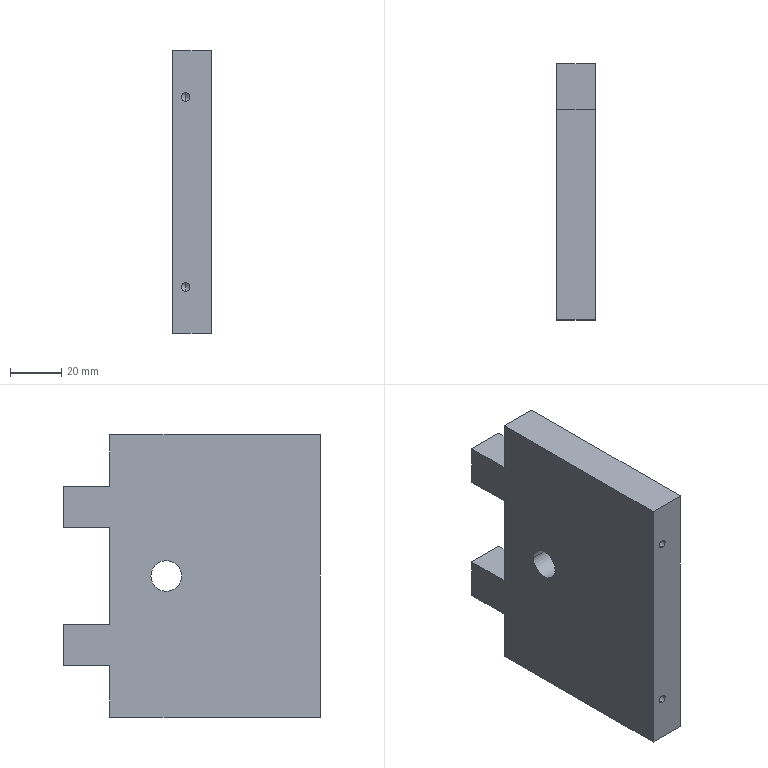Component | SolidWorks | CS021-A10-A002-1 | 1 solid | 32 faces | box 15 x 100 x 110 mm | volume 141686 mm3 | plane 14 | cylinder 10 | cone 8 | commonest cylinder face diameters 4.2 x4 3.3 x4 12 x2 | material 45
build123d program:
from build123d import *

# Parameters (mm, degrees)
SKETCH1_2_W           = 110
SKETCH1_2_H           = 100
BOSS_EXTRUDE1_DEPTH   = 7.5
M4_TAPPED_HOLE1_D     = 3.3
M4_TAPPED_HOLE1_DEPTH = 11.5
M4_TAPPED_HOLE1_TIP   = 0.9914
SKETCH4_W             = 20
SKETCH4_H             = 18
SKETCH4_W_2           = 38
CUT_EXTRUDE1_2_DEPTH  = 76.829
M5_TAPPED_HOLE1_D     = 4.2
M5_TAPPED_HOLE1_DEPTH = 12.4
M5_TAPPED_HOLE1_TIP   = 1.262
SKETCH1_R             = 6
CUT_EXTRUDE1_DEPTH    = 76.829


with BuildPart() as part:
    # Sketch1_2 → Boss-Extrude1 (new, symmetric)
    with BuildSketch(Plane(origin=(0, 0, 0), x_dir=(1, 0, 0), z_dir=(0, 1, 0))):
        Rectangle(SKETCH1_2_W, SKETCH1_2_H)
    extrude(amount=BOSS_EXTRUDE1_DEPTH, both=True)

    # M4 Tapped Hole1
    with Locations(Plane.XY.offset(50)):
        with Locations((-37, 2.5), (37, 2.5)):
            Hole(M4_TAPPED_HOLE1_D / 2, depth=M4_TAPPED_HOLE1_DEPTH)
            with Locations((0, 0, -(M4_TAPPED_HOLE1_DEPTH + M4_TAPPED_HOLE1_TIP / 2))):  # 118° drill point
                Cone(0, M4_TAPPED_HOLE1_D / 2, M4_TAPPED_HOLE1_TIP, mode=Mode.SUBTRACT)

    # Sketch4 → Cut-Extrude1_2 (cut, through all)
    with BuildSketch(Plane(origin=(0, 7.5, 0), x_dir=(1, 0, 0), z_dir=(0, 1, 0))):
        with Locations((-45, 41)):
            Rectangle(SKETCH4_W, SKETCH4_H)
        with Locations((0, 41)):
            Rectangle(SKETCH4_W_2, SKETCH4_H)
        with Locations((45, 41)):
            Rectangle(SKETCH4_W, SKETCH4_H)
    extrude(amount=-CUT_EXTRUDE1_2_DEPTH, mode=Mode.SUBTRACT)

    # M5 Tapped Hole1
    with Locations(Plane.ZY.offset(55)):
        with Locations((30, 0), (5, 0)):
            Hole(M5_TAPPED_HOLE1_D / 2, depth=M5_TAPPED_HOLE1_DEPTH)
            with Locations((0, 0, -(M5_TAPPED_HOLE1_DEPTH + M5_TAPPED_HOLE1_TIP / 2))):  # 118° drill point
                Cone(0, M5_TAPPED_HOLE1_D / 2, M5_TAPPED_HOLE1_TIP, mode=Mode.SUBTRACT)

    # Sketch1 → Cut-Extrude1 (cut, through all)
    with BuildSketch(Plane(origin=(0, 7.5, 0), x_dir=(1, 0, 0), z_dir=(0, 1, 0))):
        with Locations(Location((0, 10, 0), (0, 0, 270))):
            Circle(SKETCH1_R)
    extrude(amount=-CUT_EXTRUDE1_DEPTH, mode=Mode.SUBTRACT)


solid = part.part

# Placed as in the assembly
solid = solid.moved(Location((228.449, 74.817, 0), (90, 0, 90)))
STEP:
#1=COLOUR_RGB('',0.7922,0.8196,0.9333);
#2=FILL_AREA_STYLE_COLOUR('',#1);
#3=FILL_AREA_STYLE('',(#2));
#4=SURFACE_STYLE_FILL_AREA(#3);
#5=SURFACE_SIDE_STYLE('',(#4));
#6=SURFACE_STYLE_USAGE(.BOTH.,#5);
#7=PRESENTATION_STYLE_ASSIGNMENT((#6));
#8=CARTESIAN_POINT('',(9.289,3.575,0.));
#9=VERTEX_POINT('',#8);
#10=CARTESIAN_POINT('',(9.289,3.103,0.));
#11=VERTEX_POINT('',#10);
#12=CARTESIAN_POINT('',(9.289,3.339,0.));
#13=DIRECTION('',(-1.,0.,-0.));
#14=DIRECTION('',(0.,-1.,0.));
#15=AXIS2_PLACEMENT_3D('',#12,#13,#14);
#16=CIRCLE('',#15,0.2362);
#17=EDGE_CURVE('',#9,#11,#16,.T.);
#18=ORIENTED_EDGE('',*,*,#17,.F.);
#19=CARTESIAN_POINT('',(8.699,3.575,0.));
#20=VERTEX_POINT('',#19);
#21=CARTESIAN_POINT('',(9.289,3.575,0.));
#22=DIRECTION('',(-1.,0.,-0.));
#23=VECTOR('',#22,39.37);
#24=LINE('',#21,#23);
#25=EDGE_CURVE('',#9,#20,#24,.T.);
#26=ORIENTED_EDGE('',*,*,#25,.T.);
#27=CARTESIAN_POINT('',(8.699,3.103,-0.));
#28=VERTEX_POINT('',#27);
#29=CARTESIAN_POINT('',(8.699,3.339,-0.));
#30=DIRECTION('',(-1.,0.,-0.));
#31=DIRECTION('',(0.,-1.,0.));
#32=AXIS2_PLACEMENT_3D('',#29,#30,#31);
#33=CIRCLE('',#32,0.2362);
#34=EDGE_CURVE('',#20,#28,#33,.T.);
#35=ORIENTED_EDGE('',*,*,#34,.T.);
#36=CARTESIAN_POINT('',(9.289,3.103,0.));
#37=DIRECTION('',(-1.,0.,-0.));
#38=VECTOR('',#37,39.37);
#39=LINE('',#36,#38);
#40=EDGE_CURVE('',#11,#28,#39,.T.);
#41=ORIENTED_EDGE('',*,*,#40,.F.);
#42=EDGE_LOOP('',(#18,#26,#35,#41));
#43=FACE_OUTER_BOUND('',#42,.T.);
#44=CARTESIAN_POINT('',(9.289,3.339,0.));
#45=DIRECTION('',(-1.,0.,-0.));
#46=DIRECTION('',(0.,-1.,0.));
#47=AXIS2_PLACEMENT_3D('',#44,#45,#46);
#48=CYLINDRICAL_SURFACE('',#47,0.2362);
#49=ADVANCED_FACE('',(#43),#48,.F.);
#50=CARTESIAN_POINT('',(8.994,1.847,-1.677));
#51=VERTEX_POINT('',#50);
#52=CARTESIAN_POINT('',(8.994,1.682,-1.677));
#53=VERTEX_POINT('',#52);
#54=CARTESIAN_POINT('',(8.994,1.764,-1.677));
#55=DIRECTION('',(0.,-0.,-1.));
#56=DIRECTION('',(0.,-1.,0.));
#57=AXIS2_PLACEMENT_3D('',#54,#55,#56);
#58=CIRCLE('',#57,0.08268);
#59=EDGE_CURVE('',#51,#53,#58,.T.);
#60=ORIENTED_EDGE('',*,*,#59,.F.);
#61=CARTESIAN_POINT('',(8.994,1.847,-2.165));
#62=VERTEX_POINT('',#61);
#63=CARTESIAN_POINT('',(8.994,1.847,-2.165));
#64=DIRECTION('',(0.,-0.,-1.));
#65=VECTOR('',#64,39.37);
#66=LINE('',#63,#65);
#67=EDGE_CURVE('',#51,#62,#66,.T.);
#68=ORIENTED_EDGE('',*,*,#67,.T.);
#69=CARTESIAN_POINT('',(8.994,1.682,-2.165));
#70=VERTEX_POINT('',#69);
#71=CARTESIAN_POINT('',(8.994,1.764,-2.165));
#72=DIRECTION('',(0.,-0.,-1.));
#73=DIRECTION('',(0.,-1.,0.));
#74=AXIS2_PLACEMENT_3D('',#71,#72,#73);
#75=CIRCLE('',#74,0.08268);
#76=EDGE_CURVE('',#62,#70,#75,.T.);
#77=ORIENTED_EDGE('',*,*,#76,.T.);
#78=CARTESIAN_POINT('',(8.994,1.682,-2.165));
#79=DIRECTION('',(0.,-0.,-1.));
#80=VECTOR('',#79,39.37);
#81=LINE('',#78,#80);
#82=EDGE_CURVE('',#53,#70,#81,.T.);
#83=ORIENTED_EDGE('',*,*,#82,.F.);
#84=EDGE_LOOP('',(#60,#68,#77,#83));
#85=FACE_OUTER_BOUND('',#84,.T.);
#86=CARTESIAN_POINT('',(8.994,1.764,-2.165));
#87=DIRECTION('',(0.,-0.,-1.));
#88=DIRECTION('',(0.,-1.,0.));
#89=AXIS2_PLACEMENT_3D('',#86,#87,#88);
#90=CYLINDRICAL_SURFACE('',#89,0.08268);
#91=ADVANCED_FACE('',(#85),#90,.F.);
#92=CARTESIAN_POINT('',(8.994,1.764,-1.627));
#93=VERTEX_POINT('',#92);
#94=CARTESIAN_POINT('',(8.994,1.682,-1.677));
#95=DIRECTION('',(0.,-0.8572,-0.515));
#96=VECTOR('',#95,39.37);
#97=LINE('',#94,#96);
#98=EDGE_CURVE('',#93,#53,#97,.T.);
#99=ORIENTED_EDGE('',*,*,#98,.F.);
#100=CARTESIAN_POINT('',(8.994,1.847,-1.677));
#101=DIRECTION('',(-0.,0.8572,-0.515));
#102=VECTOR('',#101,39.37);
#103=LINE('',#100,#102);
#104=EDGE_CURVE('',#93,#51,#103,.T.);
#105=ORIENTED_EDGE('',*,*,#104,.T.);
#106=ORIENTED_EDGE('',*,*,#59,.T.);
#107=EDGE_LOOP('',(#99,#105,#106));
#108=FACE_OUTER_BOUND('',#107,.T.);
#109=CARTESIAN_POINT('',(8.994,1.764,-1.677));
#110=DIRECTION('',(0.,-0.,-1.));
#111=DIRECTION('',(0.,-1.,0.));
#112=AXIS2_PLACEMENT_3D('',#109,#110,#111);
#113=CONICAL_SURFACE('',#112,0.08268,1.03);
#114=ADVANCED_FACE('',(#108),#113,.F.);
#115=CARTESIAN_POINT('',(8.994,2.831,-1.677));
#116=VERTEX_POINT('',#115);
#117=CARTESIAN_POINT('',(8.994,2.666,-1.677));
#118=VERTEX_POINT('',#117);
#119=CARTESIAN_POINT('',(8.994,2.749,-1.677));
#120=DIRECTION('',(0.,-0.,-1.));
#121=DIRECTION('',(0.,-1.,0.));
#122=AXIS2_PLACEMENT_3D('',#119,#120,#121);
#123=CIRCLE('',#122,0.08268);
#124=EDGE_CURVE('',#116,#118,#123,.T.);
#125=ORIENTED_EDGE('',*,*,#124,.F.);
#126=CARTESIAN_POINT('',(8.994,2.831,-2.165));
#127=VERTEX_POINT('',#126);
#128=CARTESIAN_POINT('',(8.994,2.831,-2.165));
#129=DIRECTION('',(0.,-0.,-1.));
#130=VECTOR('',#129,39.37);
#131=LINE('',#128,#130);
#132=EDGE_CURVE('',#116,#127,#131,.T.);
#133=ORIENTED_EDGE('',*,*,#132,.T.);
#134=CARTESIAN_POINT('',(8.994,2.666,-2.165));
#135=VERTEX_POINT('',#134);
#136=CARTESIAN_POINT('',(8.994,2.749,-2.165));
#137=DIRECTION('',(0.,-0.,-1.));
#138=DIRECTION('',(0.,-1.,0.));
#139=AXIS2_PLACEMENT_3D('',#136,#137,#138);
#140=CIRCLE('',#139,0.08268);
#141=EDGE_CURVE('',#127,#135,#140,.T.);
#142=ORIENTED_EDGE('',*,*,#141,.T.);
#143=CARTESIAN_POINT('',(8.994,2.666,-2.165));
#144=DIRECTION('',(0.,-0.,-1.));
#145=VECTOR('',#144,39.37);
#146=LINE('',#143,#145);
#147=EDGE_CURVE('',#118,#135,#146,.T.);
#148=ORIENTED_EDGE('',*,*,#147,.F.);
#149=EDGE_LOOP('',(#125,#133,#142,#148));
#150=FACE_OUTER_BOUND('',#149,.T.);
#151=CARTESIAN_POINT('',(8.994,2.749,-2.165));
#152=DIRECTION('',(0.,-0.,-1.));
#153=DIRECTION('',(0.,-1.,0.));
#154=AXIS2_PLACEMENT_3D('',#151,#152,#153);
#155=CYLINDRICAL_SURFACE('',#154,0.08268);
#156=ADVANCED_FACE('',(#150),#155,.F.);
#157=CARTESIAN_POINT('',(8.994,2.749,-1.627));
#158=VERTEX_POINT('',#157);
#159=CARTESIAN_POINT('',(8.994,2.666,-1.677));
#160=DIRECTION('',(0.,-0.8572,-0.515));
#161=VECTOR('',#160,39.37);
#162=LINE('',#159,#161);
#163=EDGE_CURVE('',#158,#118,#162,.T.);
#164=ORIENTED_EDGE('',*,*,#163,.F.);
#165=CARTESIAN_POINT('',(8.994,2.831,-1.677));
#166=DIRECTION('',(-0.,0.8572,-0.515));
#167=VECTOR('',#166,39.37);
#168=LINE('',#165,#167);
#169=EDGE_CURVE('',#158,#116,#168,.T.);
#170=ORIENTED_EDGE('',*,*,#169,.T.);
#171=ORIENTED_EDGE('',*,*,#124,.T.);
#172=EDGE_LOOP('',(#164,#170,#171));
#173=FACE_OUTER_BOUND('',#172,.T.);
#174=CARTESIAN_POINT('',(8.994,2.749,-1.677));
#175=DIRECTION('',(0.,-0.,-1.));
#176=DIRECTION('',(0.,-1.,0.));
#177=AXIS2_PLACEMENT_3D('',#174,#175,#176);
#178=CONICAL_SURFACE('',#177,0.08268,1.03);
#179=ADVANCED_FACE('',(#173),#178,.F.);
#180=CARTESIAN_POINT('',(8.896,1.43,-1.522));
#181=VERTEX_POINT('',#180);
#182=CARTESIAN_POINT('',(8.896,1.43,-1.392));
#183=VERTEX_POINT('',#182);
#184=CARTESIAN_POINT('',(8.896,1.43,-1.457));
#185=DIRECTION('',(0.,-1.,0.));
#186=DIRECTION('',(0.,0.,1.));
#187=AXIS2_PLACEMENT_3D('',#184,#185,#186);
#188=CIRCLE('',#187,0.06496);
#189=EDGE_CURVE('',#181,#183,#188,.T.);
#190=ORIENTED_EDGE('',*,*,#189,.F.);
#191=CARTESIAN_POINT('',(8.896,0.977,-1.522));
#192=VERTEX_POINT('',#191);
#193=CARTESIAN_POINT('',(8.896,0.977,-1.522));
#194=DIRECTION('',(0.,-1.,0.));
#195=VECTOR('',#194,39.37);
#196=LINE('',#193,#195);
#197=EDGE_CURVE('',#181,#192,#196,.T.);
#198=ORIENTED_EDGE('',*,*,#197,.T.);
#199=CARTESIAN_POINT('',(8.896,0.977,-1.392));
#200=VERTEX_POINT('',#199);
#201=CARTESIAN_POINT('',(8.896,0.977,-1.457));
#202=DIRECTION('',(0.,-1.,0.));
#203=DIRECTION('',(0.,0.,1.));
#204=AXIS2_PLACEMENT_3D('',#201,#202,#203);
#205=CIRCLE('',#204,0.06496);
#206=EDGE_CURVE('',#192,#200,#205,.T.);
#207=ORIENTED_EDGE('',*,*,#206,.T.);
#208=CARTESIAN_POINT('',(8.896,0.977,-1.392));
#209=DIRECTION('',(0.,-1.,0.));
#210=VECTOR('',#209,39.37);
#211=LINE('',#208,#210);
#212=EDGE_CURVE('',#183,#200,#211,.T.);
#213=ORIENTED_EDGE('',*,*,#212,.F.);
#214=EDGE_LOOP('',(#190,#198,#207,#213));
#215=FACE_OUTER_BOUND('',#214,.T.);
#216=CARTESIAN_POINT('',(8.896,0.977,-1.457));
#217=DIRECTION('',(0.,-1.,0.));
#218=DIRECTION('',(0.,0.,1.));
#219=AXIS2_PLACEMENT_3D('',#216,#217,#218);
#220=CYLINDRICAL_SURFACE('',#219,0.06496);
#221=ADVANCED_FACE('',(#215),#220,.F.);
#222=CARTESIAN_POINT('',(8.896,1.469,-1.457));
#223=VERTEX_POINT('',#222);
#224=CARTESIAN_POINT('',(8.896,1.43,-1.392));
#225=DIRECTION('',(0.,-0.515,0.8572));
#226=VECTOR('',#225,39.37);
#227=LINE('',#224,#226);
#228=EDGE_CURVE('',#223,#183,#227,.T.);
#229=ORIENTED_EDGE('',*,*,#228,.F.);
#230=CARTESIAN_POINT('',(8.896,1.43,-1.522));
#231=DIRECTION('',(-0.,-0.515,-0.8572));
#232=VECTOR('',#231,39.37);
#233=LINE('',#230,#232);
#234=EDGE_CURVE('',#223,#181,#233,.T.);
#235=ORIENTED_EDGE('',*,*,#234,.T.);
#236=ORIENTED_EDGE('',*,*,#189,.T.);
#237=EDGE_LOOP('',(#229,#235,#236));
#238=FACE_OUTER_BOUND('',#237,.T.);
#239=CARTESIAN_POINT('',(8.896,1.43,-1.457));
#240=DIRECTION('',(0.,-1.,0.));
#241=DIRECTION('',(0.,0.,1.));
#242=AXIS2_PLACEMENT_3D('',#239,#240,#241);
#243=CONICAL_SURFACE('',#242,0.06496,1.03);
#244=ADVANCED_FACE('',(#238),#243,.F.);
#245=CARTESIAN_POINT('',(8.896,1.43,1.392));
#246=VERTEX_POINT('',#245);
#247=CARTESIAN_POINT('',(8.896,1.43,1.522));
#248=VERTEX_POINT('',#247);
#249=CARTESIAN_POINT('',(8.896,1.43,1.457));
#250=DIRECTION('',(0.,-1.,0.));
#251=DIRECTION('',(0.,0.,1.));
#252=AXIS2_PLACEMENT_3D('',#249,#250,#251);
#253=CIRCLE('',#252,0.06496);
#254=EDGE_CURVE('',#246,#248,#253,.T.);
#255=ORIENTED_EDGE('',*,*,#254,.F.);
#256=CARTESIAN_POINT('',(8.896,0.977,1.392));
#257=VERTEX_POINT('',#256);
#258=CARTESIAN_POINT('',(8.896,0.977,1.392));
#259=DIRECTION('',(0.,-1.,0.));
#260=VECTOR('',#259,39.37);
#261=LINE('',#258,#260);
#262=EDGE_CURVE('',#246,#257,#261,.T.);
#263=ORIENTED_EDGE('',*,*,#262,.T.);
#264=CARTESIAN_POINT('',(8.896,0.977,1.522));
#265=VERTEX_POINT('',#264);
#266=CARTESIAN_POINT('',(8.896,0.977,1.457));
#267=DIRECTION('',(0.,-1.,0.));
#268=DIRECTION('',(0.,0.,1.));
#269=AXIS2_PLACEMENT_3D('',#266,#267,#268);
#270=CIRCLE('',#269,0.06496);
#271=EDGE_CURVE('',#257,#265,#270,.T.);
#272=ORIENTED_EDGE('',*,*,#271,.T.);
#273=CARTESIAN_POINT('',(8.896,0.977,1.522));
#274=DIRECTION('',(0.,-1.,0.));
#275=VECTOR('',#274,39.37);
#276=LINE('',#273,#275);
#277=EDGE_CURVE('',#248,#265,#276,.T.);
#278=ORIENTED_EDGE('',*,*,#277,.F.);
#279=EDGE_LOOP('',(#255,#263,#272,#278));
#280=FACE_OUTER_BOUND('',#279,.T.);
#281=CARTESIAN_POINT('',(8.896,0.977,1.457));
#282=DIRECTION('',(0.,-1.,0.));
#283=DIRECTION('',(0.,0.,1.));
#284=AXIS2_PLACEMENT_3D('',#281,#282,#283);
#285=CYLINDRICAL_SURFACE('',#284,0.06496);
#286=ADVANCED_FACE('',(#280),#285,.F.);
#287=CARTESIAN_POINT('',(8.896,1.469,1.457));
#288=VERTEX_POINT('',#287);
#289=CARTESIAN_POINT('',(8.896,1.43,1.522));
#290=DIRECTION('',(0.,-0.515,0.8572));
#291=VECTOR('',#290,39.37);
#292=LINE('',#289,#291);
#293=EDGE_CURVE('',#288,#248,#292,.T.);
#294=ORIENTED_EDGE('',*,*,#293,.F.);
#295=CARTESIAN_POINT('',(8.896,1.43,1.392));
#296=DIRECTION('',(-0.,-0.515,-0.8572));
#297=VECTOR('',#296,39.37);
#298=LINE('',#295,#297);
#299=EDGE_CURVE('',#288,#246,#298,.T.);
#300=ORIENTED_EDGE('',*,*,#299,.T.);
#301=ORIENTED_EDGE('',*,*,#254,.T.);
#302=EDGE_LOOP('',(#294,#300,#301));
#303=FACE_OUTER_BOUND('',#302,.T.);
#304=CARTESIAN_POINT('',(8.896,1.43,1.457));
#305=DIRECTION('',(0.,-1.,0.));
#306=DIRECTION('',(0.,0.,1.));
#307=AXIS2_PLACEMENT_3D('',#304,#305,#306);
#308=CONICAL_SURFACE('',#307,0.06496,1.03);
#309=ADVANCED_FACE('',(#303),#308,.F.);
#310=CARTESIAN_POINT('',(8.699,4.914,-0.748));
#311=VERTEX_POINT('',#310);
#312=CARTESIAN_POINT('',(8.699,4.914,-1.378));
#313=VERTEX_POINT('',#312);
#314=CARTESIAN_POINT('',(8.699,4.914,-2.165));
#315=DIRECTION('',(0.,-0.,-1.));
#316=VECTOR('',#315,39.37);
#317=LINE('',#314,#316);
#318=EDGE_CURVE('',#311,#313,#317,.T.);
#319=ORIENTED_EDGE('',*,*,#318,.F.);
#320=CARTESIAN_POINT('',(9.289,4.914,-0.748));
#321=VERTEX_POINT('',#320);
#322=CARTESIAN_POINT('',(9.289,4.914,-0.748));
#323=DIRECTION('',(-1.,0.,-0.));
#324=VECTOR('',#323,39.37);
#325=LINE('',#322,#324);
#326=EDGE_CURVE('',#321,#311,#325,.T.);
#327=ORIENTED_EDGE('',*,*,#326,.F.);
#328=CARTESIAN_POINT('',(9.289,4.914,-1.378));
#329=VERTEX_POINT('',#328);
#330=CARTESIAN_POINT('',(9.289,4.914,-2.165));
#331=DIRECTION('',(0.,-0.,-1.));
#332=VECTOR('',#331,39.37);
#333=LINE('',#330,#332);
#334=EDGE_CURVE('',#321,#329,#333,.T.);
#335=ORIENTED_EDGE('',*,*,#334,.T.);
#336=CARTESIAN_POINT('',(9.289,4.914,-1.378));
#337=DIRECTION('',(-1.,0.,-0.));
#338=VECTOR('',#337,39.37);
#339=LINE('',#336,#338);
#340=EDGE_CURVE('',#329,#313,#339,.T.);
#341=ORIENTED_EDGE('',*,*,#340,.T.);
#342=EDGE_LOOP('',(#319,#327,#335,#341));
#343=FACE_OUTER_BOUND('',#342,.T.);
#344=CARTESIAN_POINT('',(8.699,4.914,-2.165));
#345=DIRECTION('',(0.,-1.,0.));
#346=DIRECTION('',(0.,0.,1.));
#347=AXIS2_PLACEMENT_3D('',#344,#345,#346);
#348=PLANE('',#347);
#349=ADVANCED_FACE('',(#343),#348,.F.);
#350=CARTESIAN_POINT('',(9.289,0.977,2.165));
#351=VERTEX_POINT('',#350);
#352=CARTESIAN_POINT('',(9.289,4.205,2.165));
#353=VERTEX_POINT('',#352);
#354=CARTESIAN_POINT('',(9.289,0.977,2.165));
#355=DIRECTION('',(-0.,1.,-0.));
#356=VECTOR('',#355,39.37);
#357=LINE('',#354,#356);
#358=EDGE_CURVE('',#351,#353,#357,.T.);
#359=ORIENTED_EDGE('',*,*,#358,.T.);
#360=CARTESIAN_POINT('',(8.699,4.205,2.165));
#361=VERTEX_POINT('',#360);
#362=CARTESIAN_POINT('',(9.289,4.205,2.165));
#363=DIRECTION('',(-1.,0.,-0.));
#364=VECTOR('',#363,39.37);
#365=LINE('',#362,#364);
#366=EDGE_CURVE('',#353,#361,#365,.T.);
#367=ORIENTED_EDGE('',*,*,#366,.T.);
#368=CARTESIAN_POINT('',(8.699,0.977,2.165));
#369=VERTEX_POINT('',#368);
#370=CARTESIAN_POINT('',(8.699,0.977,2.165));
#371=DIRECTION('',(-0.,1.,-0.));
#372=VECTOR('',#371,39.37);
#373=LINE('',#370,#372);
#374=EDGE_CURVE('',#369,#361,#373,.T.);
#375=ORIENTED_EDGE('',*,*,#374,.F.);
#376=CARTESIAN_POINT('',(8.699,0.977,2.165));
#377=DIRECTION('',(1.,-0.,0.));
#378=VECTOR('',#377,39.37);
#379=LINE('',#376,#378);
#380=EDGE_CURVE('',#369,#351,#379,.T.);
#381=ORIENTED_EDGE('',*,*,#380,.T.);
#382=EDGE_LOOP('',(#359,#367,#375,#381));
#383=FACE_OUTER_BOUND('',#382,.T.);
#384=CARTESIAN_POINT('',(8.699,0.977,2.165));
#385=DIRECTION('',(0.,-0.,-1.));
#386=DIRECTION('',(0.,-1.,0.));
#387=AXIS2_PLACEMENT_3D('',#384,#385,#386);
#388=PLANE('',#387);
#389=ADVANCED_FACE('',(#383),#388,.F.);
#390=CARTESIAN_POINT('',(8.699,4.914,1.378));
#391=VERTEX_POINT('',#390);
#392=CARTESIAN_POINT('',(8.699,4.914,0.748));
#393=VERTEX_POINT('',#392);
#394=CARTESIAN_POINT('',(8.699,4.914,-2.165));
#395=DIRECTION('',(0.,-0.,-1.));
#396=VECTOR('',#395,39.37);
#397=LINE('',#394,#396);
#398=EDGE_CURVE('',#391,#393,#397,.T.);
#399=ORIENTED_EDGE('',*,*,#398,.F.);
#400=CARTESIAN_POINT('',(9.289,4.914,1.378));
#401=VERTEX_POINT('',#400);
#402=CARTESIAN_POINT('',(9.289,4.914,1.378));
#403=DIRECTION('',(-1.,0.,-0.));
#404=VECTOR('',#403,39.37);
#405=LINE('',#402,#404);
#406=EDGE_CURVE('',#401,#391,#405,.T.);
#407=ORIENTED_EDGE('',*,*,#406,.F.);
#408=CARTESIAN_POINT('',(9.289,4.914,0.748));
#409=VERTEX_POINT('',#408);
#410=CARTESIAN_POINT('',(9.289,4.914,-2.165));
#411=DIRECTION('',(0.,-0.,-1.));
#412=VECTOR('',#411,39.37);
#413=LINE('',#410,#412);
#414=EDGE_CURVE('',#401,#409,#413,.T.);
#415=ORIENTED_EDGE('',*,*,#414,.T.);
#416=CARTESIAN_POINT('',(9.289,4.914,0.748));
#417=DIRECTION('',(-1.,0.,-0.));
#418=VECTOR('',#417,39.37);
#419=LINE('',#416,#418);
#420=EDGE_CURVE('',#409,#393,#419,.T.);
#421=ORIENTED_EDGE('',*,*,#420,.T.);
#422=EDGE_LOOP('',(#399,#407,#415,#421));
#423=FACE_OUTER_BOUND('',#422,.T.);
#424=CARTESIAN_POINT('',(8.699,4.914,-2.165));
#425=DIRECTION('',(0.,-1.,0.));
#426=DIRECTION('',(0.,0.,1.));
#427=AXIS2_PLACEMENT_3D('',#424,#425,#426);
#428=PLANE('',#427);
#429=ADVANCED_FACE('',(#423),#428,.F.);
#430=CARTESIAN_POINT('',(8.994,1.764,-2.165));
#431=DIRECTION('',(0.,-0.,-1.));
#432=DIRECTION('',(0.,-1.,0.));
#433=AXIS2_PLACEMENT_3D('',#430,#431,#432);
#434=CIRCLE('',#433,0.08268);
#435=EDGE_CURVE('',#70,#62,#434,.T.);
#436=ORIENTED_EDGE('',*,*,#435,.F.);
#437=ORIENTED_EDGE('',*,*,#76,.F.);
#438=EDGE_LOOP('',(#436,#437));
#439=FACE_BOUND('',#438,.T.);
#440=CARTESIAN_POINT('',(8.994,2.749,-2.165));
#441=DIRECTION('',(0.,-0.,-1.));
#442=DIRECTION('',(0.,-1.,0.));
#443=AXIS2_PLACEMENT_3D('',#440,#441,#442);
#444=CIRCLE('',#443,0.08268);
#445=EDGE_CURVE('',#135,#127,#444,.T.);
#446=ORIENTED_EDGE('',*,*,#445,.F.);
#447=ORIENTED_EDGE('',*,*,#141,.F.);
#448=EDGE_LOOP('',(#446,#447));
#449=FACE_BOUND('',#448,.T.);
#450=CARTESIAN_POINT('',(8.699,4.205,-2.165));
#451=VERTEX_POINT('',#450);
#452=CARTESIAN_POINT('',(8.699,0.977,-2.165));
#453=VERTEX_POINT('',#452);
#454=CARTESIAN_POINT('',(8.699,0.977,-2.165));
#455=DIRECTION('',(0.,-1.,0.));
#456=VECTOR('',#455,39.37);
#457=LINE('',#454,#456);
#458=EDGE_CURVE('',#451,#453,#457,.T.);
#459=ORIENTED_EDGE('',*,*,#458,.F.);
#460=CARTESIAN_POINT('',(9.289,4.205,-2.165));
#461=VERTEX_POINT('',#460);
#462=CARTESIAN_POINT('',(9.289,4.205,-2.165));
#463=DIRECTION('',(-1.,0.,-0.));
#464=VECTOR('',#463,39.37);
#465=LINE('',#462,#464);
#466=EDGE_CURVE('',#461,#451,#465,.T.);
#467=ORIENTED_EDGE('',*,*,#466,.F.);
#468=CARTESIAN_POINT('',(9.289,0.977,-2.165));
#469=VERTEX_POINT('',#468);
#470=CARTESIAN_POINT('',(9.289,0.977,-2.165));
#471=DIRECTION('',(0.,-1.,0.));
#472=VECTOR('',#471,39.37);
#473=LINE('',#470,#472);
#474=EDGE_CURVE('',#461,#469,#473,.T.);
#475=ORIENTED_EDGE('',*,*,#474,.T.);
#476=CARTESIAN_POINT('',(8.699,0.977,-2.165));
#477=DIRECTION('',(1.,-0.,0.));
#478=VECTOR('',#477,39.37);
#479=LINE('',#476,#478);
#480=EDGE_CURVE('',#453,#469,#479,.T.);
#481=ORIENTED_EDGE('',*,*,#480,.F.);
#482=EDGE_LOOP('',(#459,#467,#475,#481));
#483=FACE_OUTER_BOUND('',#482,.T.);
#484=CARTESIAN_POINT('',(8.699,0.977,-2.165));
#485=DIRECTION('',(-0.,0.,1.));
#486=DIRECTION('',(-0.,1.,-0.));
#487=AXIS2_PLACEMENT_3D('',#484,#485,#486);
#488=PLANE('',#487);
#489=ADVANCED_FACE('',(#439,#449,#483),#488,.F.);
#490=CARTESIAN_POINT('',(8.896,0.977,-1.457));
#491=DIRECTION('',(0.,-1.,0.));
#492=DIRECTION('',(0.,0.,1.));
#493=AXIS2_PLACEMENT_3D('',#490,#491,#492);
#494=CIRCLE('',#493,0.06496);
#495=EDGE_CURVE('',#200,#192,#494,.T.);
#496=ORIENTED_EDGE('',*,*,#495,.F.);
#497=ORIENTED_EDGE('',*,*,#206,.F.);
#498=EDGE_LOOP('',(#496,#497));
#499=FACE_BOUND('',#498,.T.);
#500=CARTESIAN_POINT('',(8.896,0.977,1.457));
#501=DIRECTION('',(0.,-1.,0.));
#502=DIRECTION('',(0.,0.,1.));
#503=AXIS2_PLACEMENT_3D('',#500,#501,#502);
#504=CIRCLE('',#503,0.06496);
#505=EDGE_CURVE('',#265,#257,#504,.T.);
#506=ORIENTED_EDGE('',*,*,#505,.F.);
#507=ORIENTED_EDGE('',*,*,#271,.F.);
#508=EDGE_LOOP('',(#506,#507));
#509=FACE_BOUND('',#508,.T.);
#510=CARTESIAN_POINT('',(9.289,0.977,-2.165));
#511=DIRECTION('',(0.,0.,1.));
#512=VECTOR('',#511,39.37);
#513=LINE('',#510,#512);
#514=EDGE_CURVE('',#469,#351,#513,.T.);
#515=ORIENTED_EDGE('',*,*,#514,.T.);
#516=ORIENTED_EDGE('',*,*,#380,.F.);
#517=CARTESIAN_POINT('',(8.699,0.977,-2.165));
#518=DIRECTION('',(0.,0.,1.));
#519=VECTOR('',#518,39.37);
#520=LINE('',#517,#519);
#521=EDGE_CURVE('',#453,#369,#520,.T.);
#522=ORIENTED_EDGE('',*,*,#521,.F.);
#523=ORIENTED_EDGE('',*,*,#480,.T.);
#524=EDGE_LOOP('',(#515,#516,#522,#523));
#525=FACE_OUTER_BOUND('',#524,.T.);
#526=CARTESIAN_POINT('',(8.699,0.977,-2.165));
#527=DIRECTION('',(-0.,1.,-0.));
#528=DIRECTION('',(0.,-0.,-1.));
#529=AXIS2_PLACEMENT_3D('',#526,#527,#528);
#530=PLANE('',#529);
#531=ADVANCED_FACE('',(#499,#509,#525),#530,.F.);
#532=CARTESIAN_POINT('',(8.699,3.339,-0.));
#533=DIRECTION('',(-1.,0.,-0.));
#534=DIRECTION('',(0.,-1.,0.));
#535=AXIS2_PLACEMENT_3D('',#532,#533,#534);
#536=CIRCLE('',#535,0.2362);
#537=EDGE_CURVE('',#28,#20,#536,.T.);
#538=ORIENTED_EDGE('',*,*,#537,.F.);
#539=ORIENTED_EDGE('',*,*,#34,.F.);
#540=EDGE_LOOP('',(#538,#539));
#541=FACE_BOUND('',#540,.T.);
#542=ORIENTED_EDGE('',*,*,#374,.T.);
#543=CARTESIAN_POINT('',(8.699,4.205,1.378));
#544=VERTEX_POINT('',#543);
#545=CARTESIAN_POINT('',(8.699,4.205,2.165));
#546=DIRECTION('',(-0.,0.,1.));
#547=VECTOR('',#546,39.37);
#548=LINE('',#545,#547);
#549=EDGE_CURVE('',#544,#361,#548,.T.);
#550=ORIENTED_EDGE('',*,*,#549,.F.);
#551=CARTESIAN_POINT('',(8.699,4.914,1.378));
#552=DIRECTION('',(0.,-1.,0.));
#553=VECTOR('',#552,39.37);
#554=LINE('',#551,#553);
#555=EDGE_CURVE('',#391,#544,#554,.T.);
#556=ORIENTED_EDGE('',*,*,#555,.F.);
#557=ORIENTED_EDGE('',*,*,#398,.T.);
#558=CARTESIAN_POINT('',(8.699,4.205,0.748));
#559=VERTEX_POINT('',#558);
#560=CARTESIAN_POINT('',(8.699,4.914,0.748));
#561=DIRECTION('',(-0.,1.,-0.));
#562=VECTOR('',#561,39.37);
#563=LINE('',#560,#562);
#564=EDGE_CURVE('',#559,#393,#563,.T.);
#565=ORIENTED_EDGE('',*,*,#564,.F.);
#566=CARTESIAN_POINT('',(8.699,4.205,-0.748));
#567=VERTEX_POINT('',#566);
#568=CARTESIAN_POINT('',(8.699,4.205,-0.748));
#569=DIRECTION('',(-0.,0.,1.));
#570=VECTOR('',#569,39.37);
#571=LINE('',#568,#570);
#572=EDGE_CURVE('',#567,#559,#571,.T.);
#573=ORIENTED_EDGE('',*,*,#572,.F.);
#574=CARTESIAN_POINT('',(8.699,4.914,-0.748));
#575=DIRECTION('',(0.,-1.,0.));
#576=VECTOR('',#575,39.37);
#577=LINE('',#574,#576);
#578=EDGE_CURVE('',#311,#567,#577,.T.);
#579=ORIENTED_EDGE('',*,*,#578,.F.);
#580=ORIENTED_EDGE('',*,*,#318,.T.);
#581=CARTESIAN_POINT('',(8.699,4.205,-1.378));
#582=VERTEX_POINT('',#581);
#583=CARTESIAN_POINT('',(8.699,4.914,-1.378));
#584=DIRECTION('',(-0.,1.,-0.));
#585=VECTOR('',#584,39.37);
#586=LINE('',#583,#585);
#587=EDGE_CURVE('',#582,#313,#586,.T.);
#588=ORIENTED_EDGE('',*,*,#587,.F.);
#589=CARTESIAN_POINT('',(8.699,4.205,-2.165));
#590=DIRECTION('',(0.,0.,1.));
#591=VECTOR('',#590,39.37);
#592=LINE('',#589,#591);
#593=EDGE_CURVE('',#451,#582,#592,.T.);
#594=ORIENTED_EDGE('',*,*,#593,.F.);
#595=ORIENTED_EDGE('',*,*,#458,.T.);
#596=ORIENTED_EDGE('',*,*,#521,.T.);
#597=EDGE_LOOP('',(#542,#550,#556,#557,#565,#573,#579,#580,#588,#594,#595,#596));
#598=FACE_OUTER_BOUND('',#597,.T.);
#599=CARTESIAN_POINT('',(8.699,2.946,0.));
#600=DIRECTION('',(1.,0.,0.));
#601=DIRECTION('',(-0.,1.,-0.));
#602=AXIS2_PLACEMENT_3D('',#599,#600,#601);
#603=PLANE('',#602);
#604=ADVANCED_FACE('',(#541,#598),#603,.F.);
#605=CARTESIAN_POINT('',(9.289,3.339,0.));
#606=DIRECTION('',(-1.,0.,-0.));
#607=DIRECTION('',(0.,-1.,0.));
#608=AXIS2_PLACEMENT_3D('',#605,#606,#607);
#609=CIRCLE('',#608,0.2362);
#610=EDGE_CURVE('',#11,#9,#609,.T.);
#611=ORIENTED_EDGE('',*,*,#610,.T.);
#612=ORIENTED_EDGE('',*,*,#17,.T.);
#613=EDGE_LOOP('',(#611,#612));
#614=FACE_BOUND('',#613,.T.);
#615=CARTESIAN_POINT('',(9.289,4.205,1.378));
#616=VERTEX_POINT('',#615);
#617=CARTESIAN_POINT('',(9.289,4.205,2.165));
#618=DIRECTION('',(-0.,0.,1.));
#619=VECTOR('',#618,39.37);
#620=LINE('',#617,#619);
#621=EDGE_CURVE('',#616,#353,#620,.T.);
#622=ORIENTED_EDGE('',*,*,#621,.T.);
#623=ORIENTED_EDGE('',*,*,#358,.F.);
#624=ORIENTED_EDGE('',*,*,#514,.F.);
#625=ORIENTED_EDGE('',*,*,#474,.F.);
#626=CARTESIAN_POINT('',(9.289,4.205,-1.378));
#627=VERTEX_POINT('',#626);
#628=CARTESIAN_POINT('',(9.289,4.205,-2.165));
#629=DIRECTION('',(0.,0.,1.));
#630=VECTOR('',#629,39.37);
#631=LINE('',#628,#630);
#632=EDGE_CURVE('',#461,#627,#631,.T.);
#633=ORIENTED_EDGE('',*,*,#632,.T.);
#634=CARTESIAN_POINT('',(9.289,4.914,-1.378));
#635=DIRECTION('',(-0.,1.,-0.));
#636=VECTOR('',#635,39.37);
#637=LINE('',#634,#636);
#638=EDGE_CURVE('',#627,#329,#637,.T.);
#639=ORIENTED_EDGE('',*,*,#638,.T.);
#640=ORIENTED_EDGE('',*,*,#334,.F.);
#641=CARTESIAN_POINT('',(9.289,4.205,-0.748));
#642=VERTEX_POINT('',#641);
#643=CARTESIAN_POINT('',(9.289,4.914,-0.748));
#644=DIRECTION('',(0.,-1.,0.));
#645=VECTOR('',#644,39.37);
#646=LINE('',#643,#645);
#647=EDGE_CURVE('',#321,#642,#646,.T.);
#648=ORIENTED_EDGE('',*,*,#647,.T.);
#649=CARTESIAN_POINT('',(9.289,4.205,0.748));
#650=VERTEX_POINT('',#649);
#651=CARTESIAN_POINT('',(9.289,4.205,-0.748));
#652=DIRECTION('',(-0.,0.,1.));
#653=VECTOR('',#652,39.37);
#654=LINE('',#651,#653);
#655=EDGE_CURVE('',#642,#650,#654,.T.);
#656=ORIENTED_EDGE('',*,*,#655,.T.);
#657=CARTESIAN_POINT('',(9.289,4.914,0.748));
#658=DIRECTION('',(-0.,1.,-0.));
#659=VECTOR('',#658,39.37);
#660=LINE('',#657,#659);
#661=EDGE_CURVE('',#650,#409,#660,.T.);
#662=ORIENTED_EDGE('',*,*,#661,.T.);
#663=ORIENTED_EDGE('',*,*,#414,.F.);
#664=CARTESIAN_POINT('',(9.289,4.914,1.378));
#665=DIRECTION('',(0.,-1.,0.));
#666=VECTOR('',#665,39.37);
#667=LINE('',#664,#666);
#668=EDGE_CURVE('',#401,#616,#667,.T.);
#669=ORIENTED_EDGE('',*,*,#668,.T.);
#670=EDGE_LOOP('',(#622,#623,#624,#625,#633,#639,#640,#648,#656,#662,#663,#669));
#671=FACE_OUTER_BOUND('',#670,.T.);
#672=CARTESIAN_POINT('',(9.289,2.946,0.));
#673=DIRECTION('',(1.,0.,0.));
#674=DIRECTION('',(-0.,1.,-0.));
#675=AXIS2_PLACEMENT_3D('',#672,#673,#674);
#676=PLANE('',#675);
#677=ADVANCED_FACE('',(#614,#671),#676,.T.);
#678=ORIENTED_EDGE('',*,*,#299,.F.);
#679=ORIENTED_EDGE('',*,*,#293,.T.);
#680=CARTESIAN_POINT('',(8.896,1.43,1.457));
#681=DIRECTION('',(0.,-1.,0.));
#682=DIRECTION('',(0.,0.,1.));
#683=AXIS2_PLACEMENT_3D('',#680,#681,#682);
#684=CIRCLE('',#683,0.06496);
#685=EDGE_CURVE('',#248,#246,#684,.T.);
#686=ORIENTED_EDGE('',*,*,#685,.T.);
#687=EDGE_LOOP('',(#678,#679,#686));
#688=FACE_OUTER_BOUND('',#687,.T.);
#689=CARTESIAN_POINT('',(8.896,1.43,1.457));
#690=DIRECTION('',(0.,-1.,0.));
#691=DIRECTION('',(0.,0.,1.));
#692=AXIS2_PLACEMENT_3D('',#689,#690,#691);
#693=CONICAL_SURFACE('',#692,0.06496,1.03);
#694=ADVANCED_FACE('',(#688),#693,.F.);
#695=ORIENTED_EDGE('',*,*,#262,.F.);
#696=ORIENTED_EDGE('',*,*,#685,.F.);
#697=ORIENTED_EDGE('',*,*,#277,.T.);
#698=ORIENTED_EDGE('',*,*,#505,.T.);
#699=EDGE_LOOP('',(#695,#696,#697,#698));
#700=FACE_OUTER_BOUND('',#699,.T.);
#701=CARTESIAN_POINT('',(8.896,0.977,1.457));
#702=DIRECTION('',(0.,-1.,0.));
#703=DIRECTION('',(0.,0.,1.));
#704=AXIS2_PLACEMENT_3D('',#701,#702,#703);
#705=CYLINDRICAL_SURFACE('',#704,0.06496);
#706=ADVANCED_FACE('',(#700),#705,.F.);
#707=ORIENTED_EDGE('',*,*,#234,.F.);
#708=ORIENTED_EDGE('',*,*,#228,.T.);
#709=CARTESIAN_POINT('',(8.896,1.43,-1.457));
#710=DIRECTION('',(0.,-1.,0.));
#711=DIRECTION('',(0.,0.,1.));
#712=AXIS2_PLACEMENT_3D('',#709,#710,#711);
#713=CIRCLE('',#712,0.06496);
#714=EDGE_CURVE('',#183,#181,#713,.T.);
#715=ORIENTED_EDGE('',*,*,#714,.T.);
#716=EDGE_LOOP('',(#707,#708,#715));
#717=FACE_OUTER_BOUND('',#716,.T.);
#718=CARTESIAN_POINT('',(8.896,1.43,-1.457));
#719=DIRECTION('',(0.,-1.,0.));
#720=DIRECTION('',(0.,0.,1.));
#721=AXIS2_PLACEMENT_3D('',#718,#719,#720);
#722=CONICAL_SURFACE('',#721,0.06496,1.03);
#723=ADVANCED_FACE('',(#717),#722,.F.);
#724=ORIENTED_EDGE('',*,*,#197,.F.);
#725=ORIENTED_EDGE('',*,*,#714,.F.);
#726=ORIENTED_EDGE('',*,*,#212,.T.);
#727=ORIENTED_EDGE('',*,*,#495,.T.);
#728=EDGE_LOOP('',(#724,#725,#726,#727));
#729=FACE_OUTER_BOUND('',#728,.T.);
#730=CARTESIAN_POINT('',(8.896,0.977,-1.457));
#731=DIRECTION('',(0.,-1.,0.));
#732=DIRECTION('',(0.,0.,1.));
#733=AXIS2_PLACEMENT_3D('',#730,#731,#732);
#734=CYLINDRICAL_SURFACE('',#733,0.06496);
#735=ADVANCED_FACE('',(#729),#734,.F.);
#736=ORIENTED_EDGE('',*,*,#587,.T.);
#737=ORIENTED_EDGE('',*,*,#340,.F.);
#738=ORIENTED_EDGE('',*,*,#638,.F.);
#739=CARTESIAN_POINT('',(9.289,4.205,-1.378));
#740=DIRECTION('',(-1.,0.,-0.));
#741=VECTOR('',#740,39.37);
#742=LINE('',#739,#741);
#743=EDGE_CURVE('',#627,#582,#742,.T.);
#744=ORIENTED_EDGE('',*,*,#743,.T.);
#745=EDGE_LOOP('',(#736,#737,#738,#744));
#746=FACE_OUTER_BOUND('',#745,.T.);
#747=CARTESIAN_POINT('',(9.289,4.914,-1.378));
#748=DIRECTION('',(-0.,0.,1.));
#749=DIRECTION('',(-0.,1.,-0.));
#750=AXIS2_PLACEMENT_3D('',#747,#748,#749);
#751=PLANE('',#750);
#752=ADVANCED_FACE('',(#746),#751,.F.);
#753=ORIENTED_EDGE('',*,*,#593,.T.);
#754=ORIENTED_EDGE('',*,*,#743,.F.);
#755=ORIENTED_EDGE('',*,*,#632,.F.);
#756=ORIENTED_EDGE('',*,*,#466,.T.);
#757=EDGE_LOOP('',(#753,#754,#755,#756));
#758=FACE_OUTER_BOUND('',#757,.T.);
#759=CARTESIAN_POINT('',(9.289,4.205,-2.165));
#760=DIRECTION('',(0.,-1.,0.));
#761=DIRECTION('',(0.,0.,1.));
#762=AXIS2_PLACEMENT_3D('',#759,#760,#761);
#763=PLANE('',#762);
#764=ADVANCED_FACE('',(#758),#763,.F.);
#765=ORIENTED_EDGE('',*,*,#578,.T.);
#766=CARTESIAN_POINT('',(9.289,4.205,-0.748));
#767=DIRECTION('',(-1.,0.,-0.));
#768=VECTOR('',#767,39.37);
#769=LINE('',#766,#768);
#770=EDGE_CURVE('',#642,#567,#769,.T.);
#771=ORIENTED_EDGE('',*,*,#770,.F.);
#772=ORIENTED_EDGE('',*,*,#647,.F.);
#773=ORIENTED_EDGE('',*,*,#326,.T.);
#774=EDGE_LOOP('',(#765,#771,#772,#773));
#775=FACE_OUTER_BOUND('',#774,.T.);
#776=CARTESIAN_POINT('',(9.289,4.914,-0.748));
#777=DIRECTION('',(0.,-0.,-1.));
#778=DIRECTION('',(0.,-1.,0.));
#779=AXIS2_PLACEMENT_3D('',#776,#777,#778);
#780=PLANE('',#779);
#781=ADVANCED_FACE('',(#775),#780,.F.);
#782=ORIENTED_EDGE('',*,*,#564,.T.);
#783=ORIENTED_EDGE('',*,*,#420,.F.);
#784=ORIENTED_EDGE('',*,*,#661,.F.);
#785=CARTESIAN_POINT('',(9.289,4.205,0.748));
#786=DIRECTION('',(-1.,0.,-0.));
#787=VECTOR('',#786,39.37);
#788=LINE('',#785,#787);
#789=EDGE_CURVE('',#650,#559,#788,.T.);
#790=ORIENTED_EDGE('',*,*,#789,.T.);
#791=EDGE_LOOP('',(#782,#783,#784,#790));
#792=FACE_OUTER_BOUND('',#791,.T.);
#793=CARTESIAN_POINT('',(9.289,4.914,0.748));
#794=DIRECTION('',(-0.,0.,1.));
#795=DIRECTION('',(-0.,1.,-0.));
#796=AXIS2_PLACEMENT_3D('',#793,#794,#795);
#797=PLANE('',#796);
#798=ADVANCED_FACE('',(#792),#797,.F.);
#799=ORIENTED_EDGE('',*,*,#572,.T.);
#800=ORIENTED_EDGE('',*,*,#789,.F.);
#801=ORIENTED_EDGE('',*,*,#655,.F.);
#802=ORIENTED_EDGE('',*,*,#770,.T.);
#803=EDGE_LOOP('',(#799,#800,#801,#802));
#804=FACE_OUTER_BOUND('',#803,.T.);
#805=CARTESIAN_POINT('',(9.289,4.205,-0.748));
#806=DIRECTION('',(0.,-1.,0.));
#807=DIRECTION('',(-0.,0.,1.));
#808=AXIS2_PLACEMENT_3D('',#805,#806,#807);
#809=PLANE('',#808);
#810=ADVANCED_FACE('',(#804),#809,.F.);
#811=ORIENTED_EDGE('',*,*,#549,.T.);
#812=ORIENTED_EDGE('',*,*,#366,.F.);
#813=ORIENTED_EDGE('',*,*,#621,.F.);
#814=CARTESIAN_POINT('',(9.289,4.205,1.378));
#815=DIRECTION('',(-1.,0.,-0.));
#816=VECTOR('',#815,39.37);
#817=LINE('',#814,#816);
#818=EDGE_CURVE('',#616,#544,#817,.T.);
#819=ORIENTED_EDGE('',*,*,#818,.T.);
#820=EDGE_LOOP('',(#811,#812,#813,#819));
#821=FACE_OUTER_BOUND('',#820,.T.);
#822=CARTESIAN_POINT('',(9.289,4.205,2.165));
#823=DIRECTION('',(0.,-1.,0.));
#824=DIRECTION('',(-0.,0.,1.));
#825=AXIS2_PLACEMENT_3D('',#822,#823,#824);
#826=PLANE('',#825);
#827=ADVANCED_FACE('',(#821),#826,.F.);
#828=ORIENTED_EDGE('',*,*,#555,.T.);
#829=ORIENTED_EDGE('',*,*,#818,.F.);
#830=ORIENTED_EDGE('',*,*,#668,.F.);
#831=ORIENTED_EDGE('',*,*,#406,.T.);
#832=EDGE_LOOP('',(#828,#829,#830,#831));
#833=FACE_OUTER_BOUND('',#832,.T.);
#834=CARTESIAN_POINT('',(9.289,4.914,1.378));
#835=DIRECTION('',(0.,-0.,-1.));
#836=DIRECTION('',(0.,-1.,0.));
#837=AXIS2_PLACEMENT_3D('',#834,#835,#836);
#838=PLANE('',#837);
#839=ADVANCED_FACE('',(#833),#838,.F.);
#840=ORIENTED_EDGE('',*,*,#169,.F.);
#841=ORIENTED_EDGE('',*,*,#163,.T.);
#842=CARTESIAN_POINT('',(8.994,2.749,-1.677));
#843=DIRECTION('',(0.,-0.,-1.));
#844=DIRECTION('',(0.,-1.,0.));
#845=AXIS2_PLACEMENT_3D('',#842,#843,#844);
#846=CIRCLE('',#845,0.08268);
#847=EDGE_CURVE('',#118,#116,#846,.T.);
#848=ORIENTED_EDGE('',*,*,#847,.T.);
#849=EDGE_LOOP('',(#840,#841,#848));
#850=FACE_OUTER_BOUND('',#849,.T.);
#851=CARTESIAN_POINT('',(8.994,2.749,-1.677));
#852=DIRECTION('',(0.,-0.,-1.));
#853=DIRECTION('',(0.,-1.,0.));
#854=AXIS2_PLACEMENT_3D('',#851,#852,#853);
#855=CONICAL_SURFACE('',#854,0.08268,1.03);
#856=ADVANCED_FACE('',(#850),#855,.F.);
#857=ORIENTED_EDGE('',*,*,#132,.F.);
#858=ORIENTED_EDGE('',*,*,#847,.F.);
#859=ORIENTED_EDGE('',*,*,#147,.T.);
#860=ORIENTED_EDGE('',*,*,#445,.T.);
#861=EDGE_LOOP('',(#857,#858,#859,#860));
#862=FACE_OUTER_BOUND('',#861,.T.);
#863=CARTESIAN_POINT('',(8.994,2.749,-2.165));
#864=DIRECTION('',(0.,-0.,-1.));
#865=DIRECTION('',(0.,-1.,0.));
#866=AXIS2_PLACEMENT_3D('',#863,#864,#865);
#867=CYLINDRICAL_SURFACE('',#866,0.08268);
#868=ADVANCED_FACE('',(#862),#867,.F.);
#869=ORIENTED_EDGE('',*,*,#104,.F.);
#870=ORIENTED_EDGE('',*,*,#98,.T.);
#871=CARTESIAN_POINT('',(8.994,1.764,-1.677));
#872=DIRECTION('',(0.,-0.,-1.));
#873=DIRECTION('',(0.,-1.,0.));
#874=AXIS2_PLACEMENT_3D('',#871,#872,#873);
#875=CIRCLE('',#874,0.08268);
#876=EDGE_CURVE('',#53,#51,#875,.T.);
#877=ORIENTED_EDGE('',*,*,#876,.T.);
#878=EDGE_LOOP('',(#869,#870,#877));
#879=FACE_OUTER_BOUND('',#878,.T.);
#880=CARTESIAN_POINT('',(8.994,1.764,-1.677));
#881=DIRECTION('',(0.,-0.,-1.));
#882=DIRECTION('',(0.,-1.,0.));
#883=AXIS2_PLACEMENT_3D('',#880,#881,#882);
#884=CONICAL_SURFACE('',#883,0.08268,1.03);
#885=ADVANCED_FACE('',(#879),#884,.F.);
#886=ORIENTED_EDGE('',*,*,#67,.F.);
#887=ORIENTED_EDGE('',*,*,#876,.F.);
#888=ORIENTED_EDGE('',*,*,#82,.T.);
#889=ORIENTED_EDGE('',*,*,#435,.T.);
#890=EDGE_LOOP('',(#886,#887,#888,#889));
#891=FACE_OUTER_BOUND('',#890,.T.);
#892=CARTESIAN_POINT('',(8.994,1.764,-2.165));
#893=DIRECTION('',(0.,-0.,-1.));
#894=DIRECTION('',(0.,-1.,0.));
#895=AXIS2_PLACEMENT_3D('',#892,#893,#894);
#896=CYLINDRICAL_SURFACE('',#895,0.08268);
#897=ADVANCED_FACE('',(#891),#896,.F.);
#898=ORIENTED_EDGE('',*,*,#25,.F.);
#899=ORIENTED_EDGE('',*,*,#610,.F.);
#900=ORIENTED_EDGE('',*,*,#40,.T.);
#901=ORIENTED_EDGE('',*,*,#537,.T.);
#902=EDGE_LOOP('',(#898,#899,#900,#901));
#903=FACE_OUTER_BOUND('',#902,.T.);
#904=CARTESIAN_POINT('',(9.289,3.339,0.));
#905=DIRECTION('',(-1.,0.,-0.));
#906=DIRECTION('',(0.,-1.,0.));
#907=AXIS2_PLACEMENT_3D('',#904,#905,#906);
#908=CYLINDRICAL_SURFACE('',#907,0.2362);
#909=ADVANCED_FACE('',(#903),#908,.F.);
#910=CLOSED_SHELL('',(#49,#91,#114,#156,#179,#221,#244,#286,#309,#349,#389,#429,#489,#531,#604,#677,#694,#706,#723,#735,#752,#764,#781,#798,#810,#827,#839,#856,#868,#885,#897,#909));
#911=MANIFOLD_SOLID_BREP('',#910);
#912=STYLED_ITEM('',(#7),#911);
#913=(LENGTH_UNIT()NAMED_UNIT(*)SI_UNIT($,.METRE.));
#914=LENGTH_MEASURE_WITH_UNIT(LENGTH_MEASURE(0.0254),#913);
#915=DIMENSIONAL_EXPONENTS(1.,0.,0.,0.,0.,0.,0.);
#916=(CONVERSION_BASED_UNIT('',#914)LENGTH_UNIT()NAMED_UNIT(#915));
#917=UNCERTAINTY_MEASURE_WITH_UNIT(LENGTH_MEASURE(0.00001),#916,'','');
#918=(NAMED_UNIT(*)PLANE_ANGLE_UNIT()SI_UNIT($,.RADIAN.));
#919=(NAMED_UNIT(*)SI_UNIT($,.STERADIAN.)SOLID_ANGLE_UNIT());
#920=(GEOMETRIC_REPRESENTATION_CONTEXT(3)GLOBAL_UNCERTAINTY_ASSIGNED_CONTEXT((#917))GLOBAL_UNIT_ASSIGNED_CONTEXT((#916,#918,#919))REPRESENTATION_CONTEXT('',''));
#921=MECHANICAL_DESIGN_GEOMETRIC_PRESENTATION_REPRESENTATION('',(#912),#920);
#922=CARTESIAN_POINT('',(0.,0.,0.));
#923=DIRECTION('',(0.,0.,1.));
#924=DIRECTION('',(1.,0.,0.));
#925=AXIS2_PLACEMENT_3D('',#922,#923,#924);
#926=(LENGTH_UNIT()NAMED_UNIT(*)SI_UNIT($,.METRE.));
#927=LENGTH_MEASURE_WITH_UNIT(LENGTH_MEASURE(0.0254),#926);
#928=DIMENSIONAL_EXPONENTS(1.,0.,0.,0.,0.,0.,0.);
#929=(CONVERSION_BASED_UNIT('',#927)LENGTH_UNIT()NAMED_UNIT(#928));
#930=UNCERTAINTY_MEASURE_WITH_UNIT(LENGTH_MEASURE(0.00001),#929,'','');
#931=(NAMED_UNIT(*)PLANE_ANGLE_UNIT()SI_UNIT($,.RADIAN.));
#932=(NAMED_UNIT(*)SI_UNIT($,.STERADIAN.)SOLID_ANGLE_UNIT());
#933=(GEOMETRIC_REPRESENTATION_CONTEXT(3)GLOBAL_UNCERTAINTY_ASSIGNED_CONTEXT((#930))GLOBAL_UNIT_ASSIGNED_CONTEXT((#929,#931,#932))REPRESENTATION_CONTEXT('',''));
#934=ADVANCED_BREP_SHAPE_REPRESENTATION('',(#911,#925),#933);
#935=PRESENTATION_LAYER_ASSIGNMENT('','',(#912));